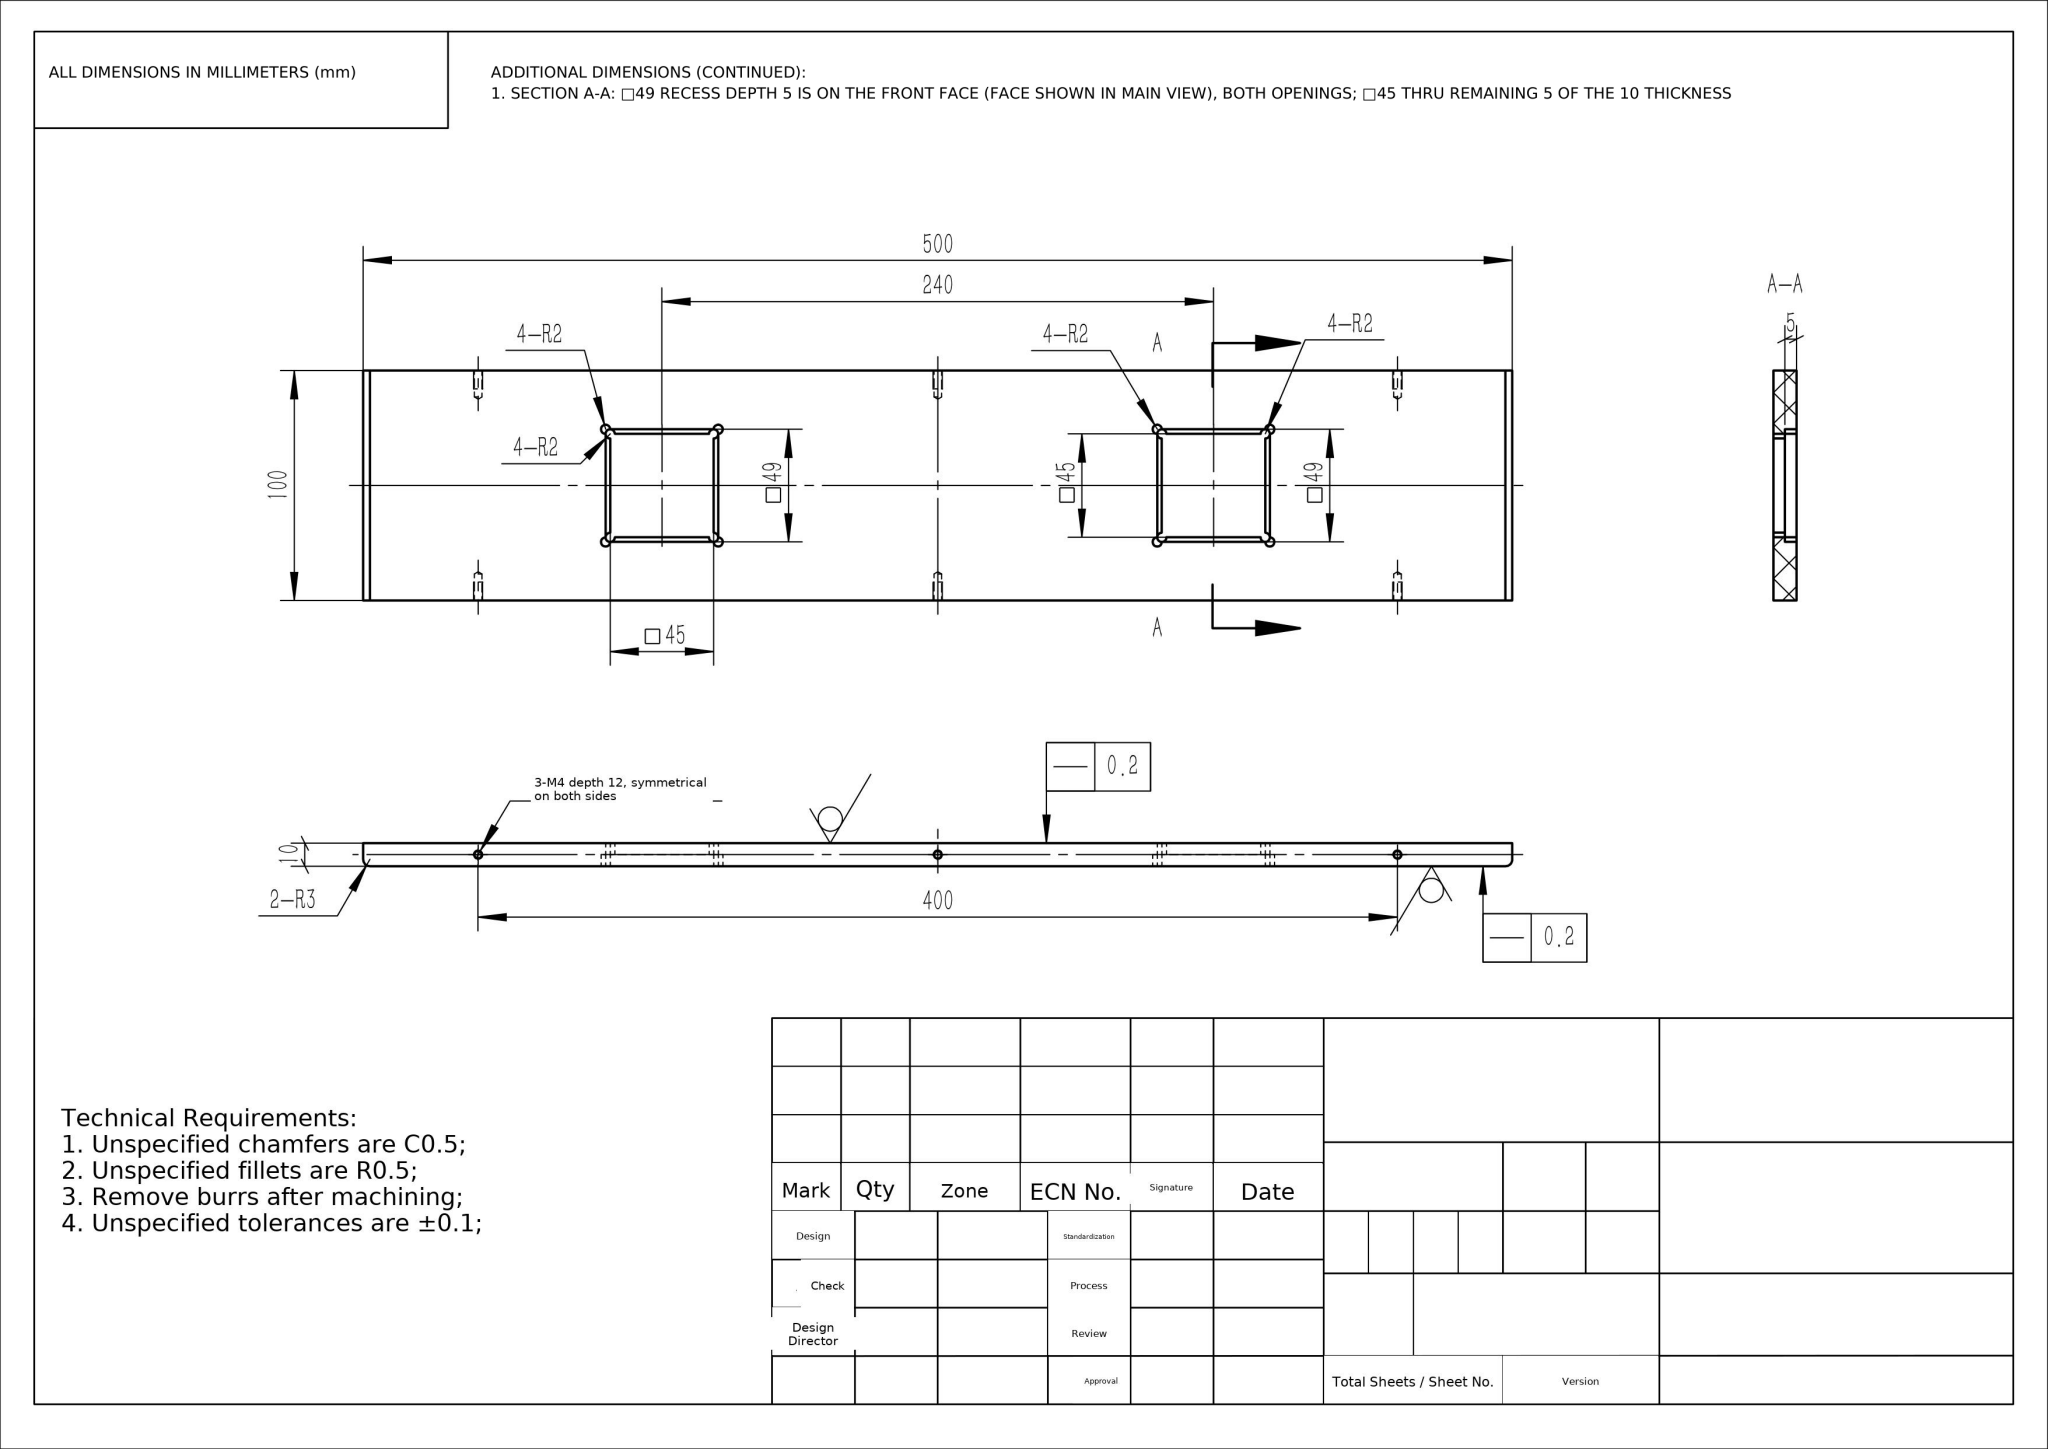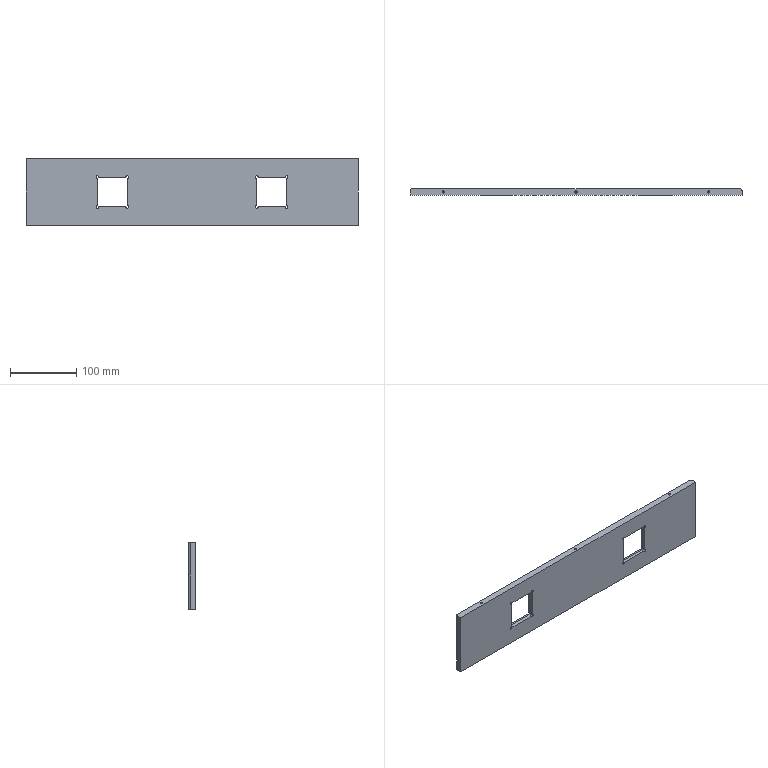Part | NX | mm | 1 solid | 88 faces | box 500 x 10 x 100 mm | volume 453993 mm3 | cylinder 38 | plane 38 | cone 12 | commonest cylinder face diameters 4 x24 3.3 x12 6 x2